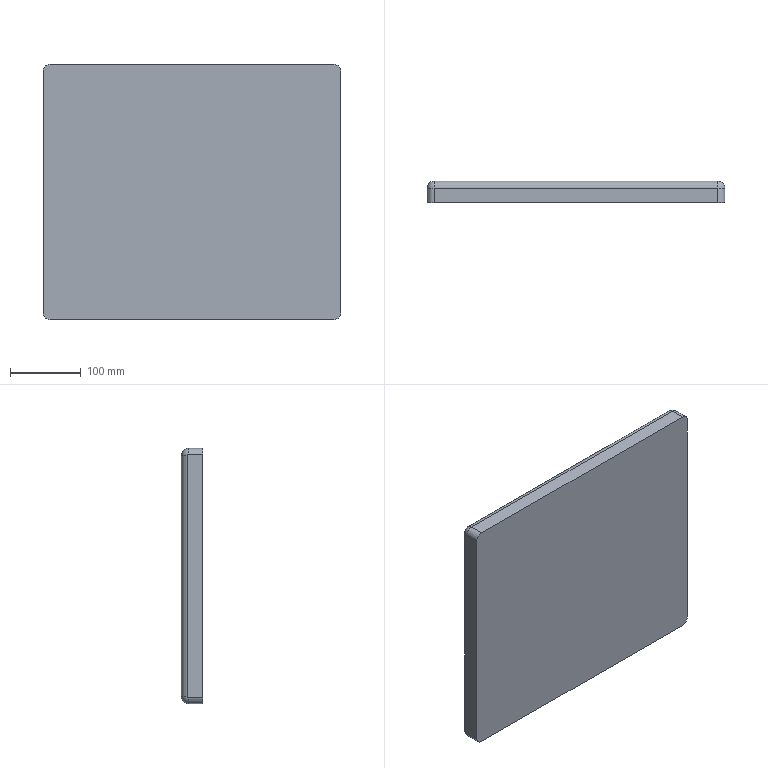Component | SolidWorks | RehabilitationChair-18-1-1 | 1 solid | 18 faces | box 419.81 x 30 x 360 mm | volume 4499203 mm3 | cylinder 8 | plane 6 | sphere 4 | commonest cylinder face diameters 20 x8
STEP:
#1=COLOUR_RGB('',0.7922,0.8196,0.9333);
#2=FILL_AREA_STYLE_COLOUR('',#1);
#3=FILL_AREA_STYLE('',(#2));
#4=SURFACE_STYLE_FILL_AREA(#3);
#5=SURFACE_SIDE_STYLE('',(#4));
#6=SURFACE_STYLE_USAGE(.BOTH.,#5);
#7=PRESENTATION_STYLE_ASSIGNMENT((#6));
#8=CARTESIAN_POINT('',(-1.582,1.912,7.087));
#9=VERTEX_POINT('',#8);
#10=CARTESIAN_POINT('',(-1.969,1.912,6.77));
#11=VERTEX_POINT('',#10);
#12=CARTESIAN_POINT('',(-1.582,1.912,6.693));
#13=DIRECTION('',(0.,-1.,0.));
#14=DIRECTION('',(0.,0.,1.));
#15=AXIS2_PLACEMENT_3D('',#12,#13,#14);
#16=CIRCLE('',#15,0.3937);
#17=EDGE_CURVE('',#9,#11,#16,.T.);
#18=ORIENTED_EDGE('',*,*,#17,.T.);
#19=CARTESIAN_POINT('',(-1.969,1.912,-6.77));
#20=VERTEX_POINT('',#19);
#21=CARTESIAN_POINT('',(-1.969,1.912,8.661));
#22=DIRECTION('',(0.,0.,-1.));
#23=VECTOR('',#22,39.37);
#24=LINE('',#21,#23);
#25=EDGE_CURVE('',#11,#20,#24,.T.);
#26=ORIENTED_EDGE('',*,*,#25,.T.);
#27=CARTESIAN_POINT('',(-1.582,1.912,-7.087));
#28=VERTEX_POINT('',#27);
#29=CARTESIAN_POINT('',(-1.582,1.912,-6.693));
#30=DIRECTION('',(0.,-1.,0.));
#31=DIRECTION('',(0.,0.,1.));
#32=AXIS2_PLACEMENT_3D('',#29,#30,#31);
#33=CIRCLE('',#32,0.3937);
#34=EDGE_CURVE('',#20,#28,#33,.T.);
#35=ORIENTED_EDGE('',*,*,#34,.T.);
#36=CARTESIAN_POINT('',(14.166,1.912,-7.087));
#37=VERTEX_POINT('',#36);
#38=CARTESIAN_POINT('',(-1.976,1.912,-7.087));
#39=DIRECTION('',(1.,0.,0.));
#40=VECTOR('',#39,39.37);
#41=LINE('',#38,#40);
#42=EDGE_CURVE('',#28,#37,#41,.T.);
#43=ORIENTED_EDGE('',*,*,#42,.T.);
#44=CARTESIAN_POINT('',(14.559,1.912,-6.693));
#45=VERTEX_POINT('',#44);
#46=CARTESIAN_POINT('',(14.166,1.912,-6.693));
#47=DIRECTION('',(0.,-1.,0.));
#48=DIRECTION('',(0.,0.,1.));
#49=AXIS2_PLACEMENT_3D('',#46,#47,#48);
#50=CIRCLE('',#49,0.3937);
#51=EDGE_CURVE('',#37,#45,#50,.T.);
#52=ORIENTED_EDGE('',*,*,#51,.T.);
#53=CARTESIAN_POINT('',(14.559,1.912,6.693));
#54=VERTEX_POINT('',#53);
#55=CARTESIAN_POINT('',(14.559,1.912,8.661));
#56=DIRECTION('',(0.,0.,-1.));
#57=VECTOR('',#56,39.37);
#58=LINE('',#55,#57);
#59=EDGE_CURVE('',#54,#45,#58,.T.);
#60=ORIENTED_EDGE('',*,*,#59,.F.);
#61=CARTESIAN_POINT('',(14.166,1.912,7.087));
#62=VERTEX_POINT('',#61);
#63=CARTESIAN_POINT('',(14.166,1.912,6.693));
#64=DIRECTION('',(0.,-1.,0.));
#65=DIRECTION('',(0.,0.,1.));
#66=AXIS2_PLACEMENT_3D('',#63,#64,#65);
#67=CIRCLE('',#66,0.3937);
#68=EDGE_CURVE('',#54,#62,#67,.T.);
#69=ORIENTED_EDGE('',*,*,#68,.T.);
#70=CARTESIAN_POINT('',(-1.976,1.912,7.087));
#71=DIRECTION('',(1.,0.,0.));
#72=VECTOR('',#71,39.37);
#73=LINE('',#70,#72);
#74=EDGE_CURVE('',#9,#62,#73,.T.);
#75=ORIENTED_EDGE('',*,*,#74,.F.);
#76=EDGE_LOOP('',(#18,#26,#35,#43,#52,#60,#69,#75));
#77=FACE_OUTER_BOUND('',#76,.T.);
#78=CARTESIAN_POINT('',(-1.976,1.912,8.661));
#79=DIRECTION('',(0.,1.,0.));
#80=DIRECTION('',(0.,0.,1.));
#81=AXIS2_PLACEMENT_3D('',#78,#79,#80);
#82=PLANE('',#81);
#83=ADVANCED_FACE('',(#77),#82,.F.);
#84=ORIENTED_EDGE('',*,*,#59,.T.);
#85=CARTESIAN_POINT('',(14.559,2.699,-6.693));
#86=VERTEX_POINT('',#85);
#87=CARTESIAN_POINT('',(14.559,3.093,-6.693));
#88=DIRECTION('',(0.,1.,0.));
#89=VECTOR('',#88,39.37);
#90=LINE('',#87,#89);
#91=EDGE_CURVE('',#45,#86,#90,.T.);
#92=ORIENTED_EDGE('',*,*,#91,.T.);
#93=CARTESIAN_POINT('',(14.559,2.699,6.693));
#94=VERTEX_POINT('',#93);
#95=CARTESIAN_POINT('',(14.559,2.699,8.661));
#96=DIRECTION('',(0.,0.,1.));
#97=VECTOR('',#96,39.37);
#98=LINE('',#95,#97);
#99=EDGE_CURVE('',#86,#94,#98,.T.);
#100=ORIENTED_EDGE('',*,*,#99,.T.);
#101=CARTESIAN_POINT('',(14.559,1.912,6.693));
#102=DIRECTION('',(0.,-1.,0.));
#103=VECTOR('',#102,39.37);
#104=LINE('',#101,#103);
#105=EDGE_CURVE('',#94,#54,#104,.T.);
#106=ORIENTED_EDGE('',*,*,#105,.T.);
#107=EDGE_LOOP('',(#84,#92,#100,#106));
#108=FACE_OUTER_BOUND('',#107,.T.);
#109=CARTESIAN_POINT('',(14.559,3.093,8.661));
#110=DIRECTION('',(-1.,0.,0.));
#111=DIRECTION('',(0.,0.,1.));
#112=AXIS2_PLACEMENT_3D('',#109,#110,#111);
#113=PLANE('',#112);
#114=ADVANCED_FACE('',(#108),#113,.F.);
#115=CARTESIAN_POINT('',(-1.582,3.093,6.693));
#116=VERTEX_POINT('',#115);
#117=CARTESIAN_POINT('',(14.166,3.093,6.693));
#118=VERTEX_POINT('',#117);
#119=CARTESIAN_POINT('',(14.559,3.093,6.693));
#120=DIRECTION('',(1.,0.,0.));
#121=VECTOR('',#120,39.37);
#122=LINE('',#119,#121);
#123=EDGE_CURVE('',#116,#118,#122,.T.);
#124=ORIENTED_EDGE('',*,*,#123,.T.);
#125=CARTESIAN_POINT('',(14.166,3.093,-6.693));
#126=VERTEX_POINT('',#125);
#127=CARTESIAN_POINT('',(14.166,3.093,8.661));
#128=DIRECTION('',(0.,0.,-1.));
#129=VECTOR('',#128,39.37);
#130=LINE('',#127,#129);
#131=EDGE_CURVE('',#118,#126,#130,.T.);
#132=ORIENTED_EDGE('',*,*,#131,.T.);
#133=CARTESIAN_POINT('',(-1.582,3.093,-6.693));
#134=VERTEX_POINT('',#133);
#135=CARTESIAN_POINT('',(-1.976,3.093,-6.693));
#136=DIRECTION('',(-1.,0.,0.));
#137=VECTOR('',#136,39.37);
#138=LINE('',#135,#137);
#139=EDGE_CURVE('',#126,#134,#138,.T.);
#140=ORIENTED_EDGE('',*,*,#139,.T.);
#141=CARTESIAN_POINT('',(-1.582,3.093,8.661));
#142=DIRECTION('',(0.,0.,1.));
#143=VECTOR('',#142,39.37);
#144=LINE('',#141,#143);
#145=EDGE_CURVE('',#134,#116,#144,.T.);
#146=ORIENTED_EDGE('',*,*,#145,.T.);
#147=EDGE_LOOP('',(#124,#132,#140,#146));
#148=FACE_OUTER_BOUND('',#147,.T.);
#149=CARTESIAN_POINT('',(-1.976,3.093,8.661));
#150=DIRECTION('',(0.,-1.,0.));
#151=DIRECTION('',(0.,0.,-1.));
#152=AXIS2_PLACEMENT_3D('',#149,#150,#151);
#153=PLANE('',#152);
#154=ADVANCED_FACE('',(#148),#153,.F.);
#155=CARTESIAN_POINT('',(14.166,2.699,7.087));
#156=VERTEX_POINT('',#155);
#157=CARTESIAN_POINT('',(-1.582,2.699,7.087));
#158=VERTEX_POINT('',#157);
#159=CARTESIAN_POINT('',(-1.976,2.699,7.087));
#160=DIRECTION('',(-1.,0.,0.));
#161=VECTOR('',#160,39.37);
#162=LINE('',#159,#161);
#163=EDGE_CURVE('',#156,#158,#162,.T.);
#164=ORIENTED_EDGE('',*,*,#163,.T.);
#165=CARTESIAN_POINT('',(-1.582,1.912,7.087));
#166=DIRECTION('',(0.,-1.,0.));
#167=VECTOR('',#166,39.37);
#168=LINE('',#165,#167);
#169=EDGE_CURVE('',#158,#9,#168,.T.);
#170=ORIENTED_EDGE('',*,*,#169,.T.);
#171=ORIENTED_EDGE('',*,*,#74,.T.);
#172=CARTESIAN_POINT('',(14.166,3.093,7.087));
#173=DIRECTION('',(0.,1.,0.));
#174=VECTOR('',#173,39.37);
#175=LINE('',#172,#174);
#176=EDGE_CURVE('',#62,#156,#175,.T.);
#177=ORIENTED_EDGE('',*,*,#176,.T.);
#178=EDGE_LOOP('',(#164,#170,#171,#177));
#179=FACE_OUTER_BOUND('',#178,.T.);
#180=CARTESIAN_POINT('',(-1.976,3.093,7.087));
#181=DIRECTION('',(0.,0.,1.));
#182=DIRECTION('',(1.,0.,0.));
#183=AXIS2_PLACEMENT_3D('',#180,#181,#182);
#184=PLANE('',#183);
#185=ADVANCED_FACE('',(#179),#184,.T.);
#186=ORIENTED_EDGE('',*,*,#42,.F.);
#187=CARTESIAN_POINT('',(-1.582,2.699,-7.087));
#188=VERTEX_POINT('',#187);
#189=CARTESIAN_POINT('',(-1.582,3.093,-7.087));
#190=DIRECTION('',(0.,1.,0.));
#191=VECTOR('',#190,39.37);
#192=LINE('',#189,#191);
#193=EDGE_CURVE('',#28,#188,#192,.T.);
#194=ORIENTED_EDGE('',*,*,#193,.T.);
#195=CARTESIAN_POINT('',(14.166,2.699,-7.087));
#196=VERTEX_POINT('',#195);
#197=CARTESIAN_POINT('',(-1.976,2.699,-7.087));
#198=DIRECTION('',(1.,0.,0.));
#199=VECTOR('',#198,39.37);
#200=LINE('',#197,#199);
#201=EDGE_CURVE('',#188,#196,#200,.T.);
#202=ORIENTED_EDGE('',*,*,#201,.T.);
#203=CARTESIAN_POINT('',(14.166,3.093,-7.087));
#204=DIRECTION('',(0.,-1.,0.));
#205=VECTOR('',#204,39.37);
#206=LINE('',#203,#205);
#207=EDGE_CURVE('',#196,#37,#206,.T.);
#208=ORIENTED_EDGE('',*,*,#207,.T.);
#209=EDGE_LOOP('',(#186,#194,#202,#208));
#210=FACE_OUTER_BOUND('',#209,.T.);
#211=CARTESIAN_POINT('',(-1.976,3.093,-7.087));
#212=DIRECTION('',(0.,0.,1.));
#213=DIRECTION('',(1.,0.,0.));
#214=AXIS2_PLACEMENT_3D('',#211,#212,#213);
#215=PLANE('',#214);
#216=ADVANCED_FACE('',(#210),#215,.F.);
#217=CARTESIAN_POINT('',(-1.969,2.699,6.77));
#218=VERTEX_POINT('',#217);
#219=CARTESIAN_POINT('',(-1.969,3.093,6.77));
#220=DIRECTION('',(0.,1.,0.));
#221=VECTOR('',#220,39.37);
#222=LINE('',#219,#221);
#223=EDGE_CURVE('',#11,#218,#222,.T.);
#224=ORIENTED_EDGE('',*,*,#223,.F.);
#225=ORIENTED_EDGE('',*,*,#17,.F.);
#226=ORIENTED_EDGE('',*,*,#169,.F.);
#227=CARTESIAN_POINT('',(-1.582,2.699,6.693));
#228=DIRECTION('',(0.,1.,0.));
#229=DIRECTION('',(0.,0.,1.));
#230=AXIS2_PLACEMENT_3D('',#227,#228,#229);
#231=CIRCLE('',#230,0.3937);
#232=EDGE_CURVE('',#218,#158,#231,.T.);
#233=ORIENTED_EDGE('',*,*,#232,.F.);
#234=EDGE_LOOP('',(#224,#225,#226,#233));
#235=FACE_OUTER_BOUND('',#234,.T.);
#236=CARTESIAN_POINT('',(-1.582,3.093,6.693));
#237=DIRECTION('',(0.,1.,0.));
#238=DIRECTION('',(0.,0.,1.));
#239=AXIS2_PLACEMENT_3D('',#236,#237,#238);
#240=CYLINDRICAL_SURFACE('',#239,0.3937);
#241=ADVANCED_FACE('',(#235),#240,.T.);
#242=CARTESIAN_POINT('',(-1.969,2.776,6.693));
#243=VERTEX_POINT('',#242);
#244=CARTESIAN_POINT('',(-1.969,2.776,-6.693));
#245=VERTEX_POINT('',#244);
#246=CARTESIAN_POINT('',(-1.969,2.776,8.661));
#247=DIRECTION('',(0.,0.,-1.));
#248=VECTOR('',#247,39.37);
#249=LINE('',#246,#248);
#250=EDGE_CURVE('',#243,#245,#249,.T.);
#251=ORIENTED_EDGE('',*,*,#250,.F.);
#252=CARTESIAN_POINT('',(-1.582,2.699,6.693));
#253=DIRECTION('',(0.,0.,1.));
#254=DIRECTION('',(1.,0.,0.));
#255=AXIS2_PLACEMENT_3D('',#252,#253,#254);
#256=CIRCLE('',#255,0.3937);
#257=EDGE_CURVE('',#116,#243,#256,.T.);
#258=ORIENTED_EDGE('',*,*,#257,.F.);
#259=ORIENTED_EDGE('',*,*,#145,.F.);
#260=CARTESIAN_POINT('',(-1.582,2.699,-6.693));
#261=DIRECTION('',(0.,0.,-1.));
#262=DIRECTION('',(-1.,0.,0.));
#263=AXIS2_PLACEMENT_3D('',#260,#261,#262);
#264=CIRCLE('',#263,0.3937);
#265=EDGE_CURVE('',#245,#134,#264,.T.);
#266=ORIENTED_EDGE('',*,*,#265,.F.);
#267=EDGE_LOOP('',(#251,#258,#259,#266));
#268=FACE_OUTER_BOUND('',#267,.T.);
#269=CARTESIAN_POINT('',(-1.582,2.699,8.661));
#270=DIRECTION('',(0.,0.,-1.));
#271=DIRECTION('',(-1.,0.,0.));
#272=AXIS2_PLACEMENT_3D('',#269,#270,#271);
#273=CYLINDRICAL_SURFACE('',#272,0.3937);
#274=ADVANCED_FACE('',(#268),#273,.T.);
#275=CARTESIAN_POINT('',(-1.969,2.699,-6.77));
#276=VERTEX_POINT('',#275);
#277=CARTESIAN_POINT('',(-1.969,3.093,-6.77));
#278=DIRECTION('',(0.,-1.,0.));
#279=VECTOR('',#278,39.37);
#280=LINE('',#277,#279);
#281=EDGE_CURVE('',#276,#20,#280,.T.);
#282=ORIENTED_EDGE('',*,*,#281,.F.);
#283=CARTESIAN_POINT('',(-1.582,2.699,-6.693));
#284=DIRECTION('',(0.,1.,0.));
#285=DIRECTION('',(0.,0.,1.));
#286=AXIS2_PLACEMENT_3D('',#283,#284,#285);
#287=CIRCLE('',#286,0.3937);
#288=EDGE_CURVE('',#188,#276,#287,.T.);
#289=ORIENTED_EDGE('',*,*,#288,.F.);
#290=ORIENTED_EDGE('',*,*,#193,.F.);
#291=ORIENTED_EDGE('',*,*,#34,.F.);
#292=EDGE_LOOP('',(#282,#289,#290,#291));
#293=FACE_OUTER_BOUND('',#292,.T.);
#294=CARTESIAN_POINT('',(-1.582,3.093,-6.693));
#295=DIRECTION('',(0.,-1.,0.));
#296=DIRECTION('',(0.,0.,-1.));
#297=AXIS2_PLACEMENT_3D('',#294,#295,#296);
#298=CYLINDRICAL_SURFACE('',#297,0.3937);
#299=ADVANCED_FACE('',(#293),#298,.T.);
#300=CARTESIAN_POINT('',(-1.969,2.699,6.693));
#301=DIRECTION('',(-1.,0.,0.));
#302=DIRECTION('',(0.,0.,-1.));
#303=AXIS2_PLACEMENT_3D('',#300,#301,#302);
#304=CIRCLE('',#303,0.0771);
#305=EDGE_CURVE('',#218,#243,#304,.T.);
#306=ORIENTED_EDGE('',*,*,#305,.F.);
#307=ORIENTED_EDGE('',*,*,#232,.T.);
#308=CARTESIAN_POINT('',(-1.582,2.699,6.693));
#309=DIRECTION('',(1.,0.,0.));
#310=DIRECTION('',(0.,0.,1.));
#311=AXIS2_PLACEMENT_3D('',#308,#309,#310);
#312=CIRCLE('',#311,0.3937);
#313=EDGE_CURVE('',#116,#158,#312,.T.);
#314=ORIENTED_EDGE('',*,*,#313,.F.);
#315=ORIENTED_EDGE('',*,*,#257,.T.);
#316=EDGE_LOOP('',(#306,#307,#314,#315));
#317=FACE_OUTER_BOUND('',#316,.T.);
#318=CARTESIAN_POINT('',(-1.582,2.699,6.693));
#319=DIRECTION('',(0.,1.,0.));
#320=DIRECTION('',(0.,0.,1.));
#321=AXIS2_PLACEMENT_3D('',#318,#319,#320);
#322=SPHERICAL_SURFACE('',#321,0.3937);
#323=ADVANCED_FACE('',(#317),#322,.T.);
#324=CARTESIAN_POINT('',(-1.969,2.699,-6.693));
#325=DIRECTION('',(-1.,0.,0.));
#326=DIRECTION('',(0.,0.,-1.));
#327=AXIS2_PLACEMENT_3D('',#324,#325,#326);
#328=CIRCLE('',#327,0.0771);
#329=EDGE_CURVE('',#245,#276,#328,.T.);
#330=ORIENTED_EDGE('',*,*,#329,.F.);
#331=ORIENTED_EDGE('',*,*,#265,.T.);
#332=CARTESIAN_POINT('',(-1.582,2.699,-6.693));
#333=DIRECTION('',(1.,0.,0.));
#334=DIRECTION('',(0.,0.,1.));
#335=AXIS2_PLACEMENT_3D('',#332,#333,#334);
#336=CIRCLE('',#335,0.3937);
#337=EDGE_CURVE('',#188,#134,#336,.T.);
#338=ORIENTED_EDGE('',*,*,#337,.F.);
#339=ORIENTED_EDGE('',*,*,#288,.T.);
#340=EDGE_LOOP('',(#330,#331,#338,#339));
#341=FACE_OUTER_BOUND('',#340,.T.);
#342=CARTESIAN_POINT('',(-1.582,2.699,-6.693));
#343=DIRECTION('',(0.,1.,0.));
#344=DIRECTION('',(-0.,0.,1.));
#345=AXIS2_PLACEMENT_3D('',#342,#343,#344);
#346=SPHERICAL_SURFACE('',#345,0.3937);
#347=ADVANCED_FACE('',(#341),#346,.T.);
#348=ORIENTED_EDGE('',*,*,#68,.F.);
#349=ORIENTED_EDGE('',*,*,#105,.F.);
#350=CARTESIAN_POINT('',(14.166,2.699,6.693));
#351=DIRECTION('',(0.,1.,0.));
#352=DIRECTION('',(0.,0.,1.));
#353=AXIS2_PLACEMENT_3D('',#350,#351,#352);
#354=CIRCLE('',#353,0.3937);
#355=EDGE_CURVE('',#156,#94,#354,.T.);
#356=ORIENTED_EDGE('',*,*,#355,.F.);
#357=ORIENTED_EDGE('',*,*,#176,.F.);
#358=EDGE_LOOP('',(#348,#349,#356,#357));
#359=FACE_OUTER_BOUND('',#358,.T.);
#360=CARTESIAN_POINT('',(14.166,3.093,6.693));
#361=DIRECTION('',(0.,-1.,0.));
#362=DIRECTION('',(0.,0.,-1.));
#363=AXIS2_PLACEMENT_3D('',#360,#361,#362);
#364=CYLINDRICAL_SURFACE('',#363,0.3937);
#365=ADVANCED_FACE('',(#359),#364,.T.);
#366=ORIENTED_EDGE('',*,*,#313,.T.);
#367=ORIENTED_EDGE('',*,*,#163,.F.);
#368=CARTESIAN_POINT('',(14.166,2.699,6.693));
#369=DIRECTION('',(1.,0.,0.));
#370=DIRECTION('',(0.,0.,-1.));
#371=AXIS2_PLACEMENT_3D('',#368,#369,#370);
#372=CIRCLE('',#371,0.3937);
#373=EDGE_CURVE('',#118,#156,#372,.T.);
#374=ORIENTED_EDGE('',*,*,#373,.F.);
#375=ORIENTED_EDGE('',*,*,#123,.F.);
#376=EDGE_LOOP('',(#366,#367,#374,#375));
#377=FACE_OUTER_BOUND('',#376,.T.);
#378=CARTESIAN_POINT('',(-1.976,2.699,6.693));
#379=DIRECTION('',(1.,0.,0.));
#380=DIRECTION('',(0.,0.,-1.));
#381=AXIS2_PLACEMENT_3D('',#378,#379,#380);
#382=CYLINDRICAL_SURFACE('',#381,0.3937);
#383=ADVANCED_FACE('',(#377),#382,.T.);
#384=ORIENTED_EDGE('',*,*,#337,.T.);
#385=ORIENTED_EDGE('',*,*,#139,.F.);
#386=CARTESIAN_POINT('',(14.166,2.699,-6.693));
#387=DIRECTION('',(1.,0.,0.));
#388=DIRECTION('',(0.,0.,-1.));
#389=AXIS2_PLACEMENT_3D('',#386,#387,#388);
#390=CIRCLE('',#389,0.3937);
#391=EDGE_CURVE('',#196,#126,#390,.T.);
#392=ORIENTED_EDGE('',*,*,#391,.F.);
#393=ORIENTED_EDGE('',*,*,#201,.F.);
#394=EDGE_LOOP('',(#384,#385,#392,#393));
#395=FACE_OUTER_BOUND('',#394,.T.);
#396=CARTESIAN_POINT('',(-1.976,2.699,-6.693));
#397=DIRECTION('',(-1.,0.,0.));
#398=DIRECTION('',(0.,0.,1.));
#399=AXIS2_PLACEMENT_3D('',#396,#397,#398);
#400=CYLINDRICAL_SURFACE('',#399,0.3937);
#401=ADVANCED_FACE('',(#395),#400,.T.);
#402=ORIENTED_EDGE('',*,*,#51,.F.);
#403=ORIENTED_EDGE('',*,*,#207,.F.);
#404=CARTESIAN_POINT('',(14.166,2.699,-6.693));
#405=DIRECTION('',(0.,1.,0.));
#406=DIRECTION('',(0.,0.,1.));
#407=AXIS2_PLACEMENT_3D('',#404,#405,#406);
#408=CIRCLE('',#407,0.3937);
#409=EDGE_CURVE('',#86,#196,#408,.T.);
#410=ORIENTED_EDGE('',*,*,#409,.F.);
#411=ORIENTED_EDGE('',*,*,#91,.F.);
#412=EDGE_LOOP('',(#402,#403,#410,#411));
#413=FACE_OUTER_BOUND('',#412,.T.);
#414=CARTESIAN_POINT('',(14.166,3.093,-6.693));
#415=DIRECTION('',(0.,1.,0.));
#416=DIRECTION('',(0.,0.,1.));
#417=AXIS2_PLACEMENT_3D('',#414,#415,#416);
#418=CYLINDRICAL_SURFACE('',#417,0.3937);
#419=ADVANCED_FACE('',(#413),#418,.T.);
#420=ORIENTED_EDGE('',*,*,#373,.T.);
#421=ORIENTED_EDGE('',*,*,#355,.T.);
#422=CARTESIAN_POINT('',(14.166,2.699,6.693));
#423=DIRECTION('',(0.,0.,-1.));
#424=DIRECTION('',(1.,0.,0.));
#425=AXIS2_PLACEMENT_3D('',#422,#423,#424);
#426=CIRCLE('',#425,0.3937);
#427=EDGE_CURVE('',#118,#94,#426,.T.);
#428=ORIENTED_EDGE('',*,*,#427,.F.);
#429=EDGE_LOOP('',(#420,#421,#428));
#430=FACE_OUTER_BOUND('',#429,.T.);
#431=CARTESIAN_POINT('',(14.166,2.699,6.693));
#432=DIRECTION('',(0.,1.,0.));
#433=DIRECTION('',(1.,0.,0.));
#434=AXIS2_PLACEMENT_3D('',#431,#432,#433);
#435=SPHERICAL_SURFACE('',#434,0.3937);
#436=ADVANCED_FACE('',(#430),#435,.T.);
#437=ORIENTED_EDGE('',*,*,#409,.T.);
#438=ORIENTED_EDGE('',*,*,#391,.T.);
#439=CARTESIAN_POINT('',(14.166,2.699,-6.693));
#440=DIRECTION('',(0.,0.,1.));
#441=DIRECTION('',(-1.,0.,0.));
#442=AXIS2_PLACEMENT_3D('',#439,#440,#441);
#443=CIRCLE('',#442,0.3937);
#444=EDGE_CURVE('',#86,#126,#443,.T.);
#445=ORIENTED_EDGE('',*,*,#444,.F.);
#446=EDGE_LOOP('',(#437,#438,#445));
#447=FACE_OUTER_BOUND('',#446,.T.);
#448=CARTESIAN_POINT('',(14.166,2.699,-6.693));
#449=DIRECTION('',(0.,1.,0.));
#450=DIRECTION('',(-1.,0.,0.));
#451=AXIS2_PLACEMENT_3D('',#448,#449,#450);
#452=SPHERICAL_SURFACE('',#451,0.3937);
#453=ADVANCED_FACE('',(#447),#452,.T.);
#454=ORIENTED_EDGE('',*,*,#427,.T.);
#455=ORIENTED_EDGE('',*,*,#99,.F.);
#456=ORIENTED_EDGE('',*,*,#444,.T.);
#457=ORIENTED_EDGE('',*,*,#131,.F.);
#458=EDGE_LOOP('',(#454,#455,#456,#457));
#459=FACE_OUTER_BOUND('',#458,.T.);
#460=CARTESIAN_POINT('',(14.166,2.699,8.661));
#461=DIRECTION('',(0.,0.,-1.));
#462=DIRECTION('',(-1.,0.,0.));
#463=AXIS2_PLACEMENT_3D('',#460,#461,#462);
#464=CYLINDRICAL_SURFACE('',#463,0.3937);
#465=ADVANCED_FACE('',(#459),#464,.T.);
#466=ORIENTED_EDGE('',*,*,#223,.T.);
#467=ORIENTED_EDGE('',*,*,#305,.T.);
#468=ORIENTED_EDGE('',*,*,#250,.T.);
#469=ORIENTED_EDGE('',*,*,#329,.T.);
#470=ORIENTED_EDGE('',*,*,#281,.T.);
#471=ORIENTED_EDGE('',*,*,#25,.F.);
#472=EDGE_LOOP('',(#466,#467,#468,#469,#470,#471));
#473=FACE_OUTER_BOUND('',#472,.T.);
#474=CARTESIAN_POINT('',(-1.969,0.,0.));
#475=DIRECTION('',(1.,0.,0.));
#476=DIRECTION('',(0.,0.,-1.));
#477=AXIS2_PLACEMENT_3D('',#474,#475,#476);
#478=PLANE('',#477);
#479=ADVANCED_FACE('',(#473),#478,.F.);
#480=CLOSED_SHELL('',(#83,#114,#154,#185,#216,#241,#274,#299,#323,#347,#365,#383,#401,#419,#436,#453,#465,#479));
#481=MANIFOLD_SOLID_BREP('',#480);
#482=STYLED_ITEM('',(#7),#481);
#483=(LENGTH_UNIT()NAMED_UNIT(*)SI_UNIT($,.METRE.));
#484=LENGTH_MEASURE_WITH_UNIT(LENGTH_MEASURE(0.0254),#483);
#485=DIMENSIONAL_EXPONENTS(1.,0.,0.,0.,0.,0.,0.);
#486=(CONVERSION_BASED_UNIT('',#484)LENGTH_UNIT()NAMED_UNIT(#485));
#487=UNCERTAINTY_MEASURE_WITH_UNIT(LENGTH_MEASURE(0.00001),#486,'','');
#488=(NAMED_UNIT(*)PLANE_ANGLE_UNIT()SI_UNIT($,.RADIAN.));
#489=(NAMED_UNIT(*)SI_UNIT($,.STERADIAN.)SOLID_ANGLE_UNIT());
#490=(GEOMETRIC_REPRESENTATION_CONTEXT(3)GLOBAL_UNCERTAINTY_ASSIGNED_CONTEXT((#487))GLOBAL_UNIT_ASSIGNED_CONTEXT((#486,#488,#489))REPRESENTATION_CONTEXT('',''));
#491=MECHANICAL_DESIGN_GEOMETRIC_PRESENTATION_REPRESENTATION('',(#482),#490);
#492=CARTESIAN_POINT('',(0.,0.,0.));
#493=DIRECTION('',(0.,0.,1.));
#494=DIRECTION('',(1.,0.,0.));
#495=AXIS2_PLACEMENT_3D('',#492,#493,#494);
#496=(LENGTH_UNIT()NAMED_UNIT(*)SI_UNIT($,.METRE.));
#497=LENGTH_MEASURE_WITH_UNIT(LENGTH_MEASURE(0.0254),#496);
#498=DIMENSIONAL_EXPONENTS(1.,0.,0.,0.,0.,0.,0.);
#499=(CONVERSION_BASED_UNIT('',#497)LENGTH_UNIT()NAMED_UNIT(#498));
#500=UNCERTAINTY_MEASURE_WITH_UNIT(LENGTH_MEASURE(0.00001),#499,'','');
#501=(NAMED_UNIT(*)PLANE_ANGLE_UNIT()SI_UNIT($,.RADIAN.));
#502=(NAMED_UNIT(*)SI_UNIT($,.STERADIAN.)SOLID_ANGLE_UNIT());
#503=(GEOMETRIC_REPRESENTATION_CONTEXT(3)GLOBAL_UNCERTAINTY_ASSIGNED_CONTEXT((#500))GLOBAL_UNIT_ASSIGNED_CONTEXT((#499,#501,#502))REPRESENTATION_CONTEXT('',''));
#504=ADVANCED_BREP_SHAPE_REPRESENTATION('',(#481,#495),#503);
#505=PRESENTATION_LAYER_ASSIGNMENT('','',(#482));